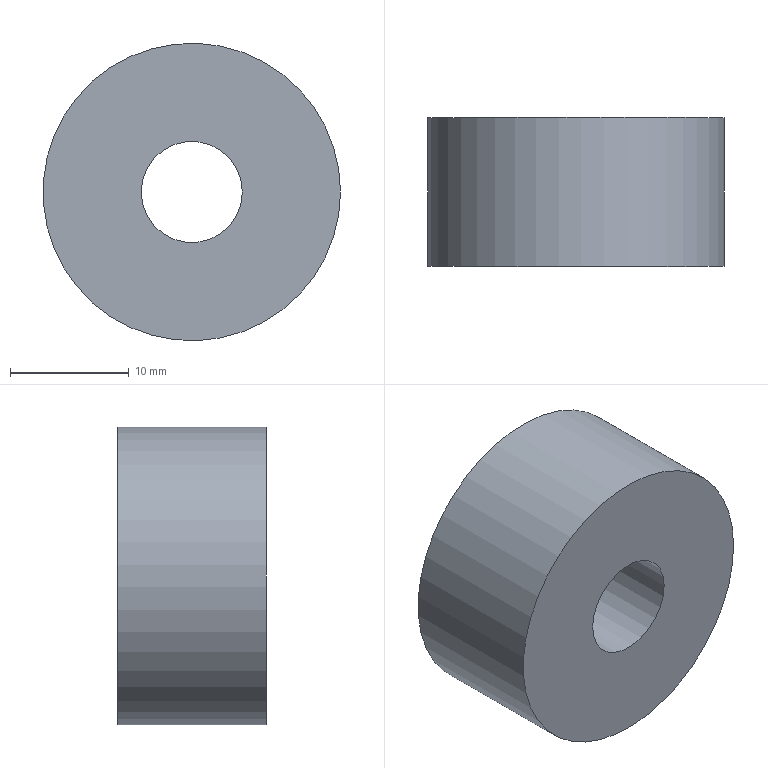Component | NX | 7_WASHER | 1 solid | 4 faces | box 25 x 12.5 x 25 mm | volume 5427 mm3 | plane 2 | cylinder 2 | commonest cylinder face diameters 25 x1 8.5 x1
STEP:
#1=CARTESIAN_POINT('',(0.,0.,0.));
#2=DIRECTION('',(0.,0.,1.));
#3=DIRECTION('',(1.,0.,0.));
#4=AXIS2_PLACEMENT_3D('',#1,#2,#3);
#5=CARTESIAN_POINT('',(6.27,26.63,14.672));
#6=VERTEX_POINT('',#5);
#7=CARTESIAN_POINT('',(2.02,26.63,14.672));
#8=DIRECTION('',(0.,-1.,0.));
#9=DIRECTION('',(1.,0.,0.));
#10=AXIS2_PLACEMENT_3D('',#7,#8,#9);
#11=CIRCLE('',#10,4.25);
#12=CARTESIAN_POINT('',(2.02,26.63,14.672));
#13=DIRECTION('',(0.,1.,0.));
#14=DIRECTION('',(1.,0.,0.));
#15=AXIS2_PLACEMENT_3D('',#12,#13,#14);
#16=PLANE('',#15);
#17=CARTESIAN_POINT('',(4.25,0.));
#18=CARTESIAN_POINT('',(4.25,-7.361));
#19=CARTESIAN_POINT('',(-2.125,-3.681));
#20=CARTESIAN_POINT('',(-8.5,-0.));
#21=CARTESIAN_POINT('',(-2.125,3.681));
#22=CARTESIAN_POINT('',(4.25,7.361));
#23=CARTESIAN_POINT('',(4.25,0.));
#24=(BOUNDED_CURVE()B_SPLINE_CURVE(2,(#17,#18,#19,#20,#21,#22,#23),.UNSPECIFIED.,.T.,.F.)B_SPLINE_CURVE_WITH_KNOTS((1,2,2,2,2,1),(-2.094,0.,2.094,4.189,6.283,8.378),.UNSPECIFIED.)CURVE()GEOMETRIC_REPRESENTATION_ITEM()RATIONAL_B_SPLINE_CURVE((1.,0.5,1.,0.5,1.,0.5,1.))REPRESENTATION_ITEM(''));
#25=(GEOMETRIC_REPRESENTATION_CONTEXT(2)PARAMETRIC_REPRESENTATION_CONTEXT()REPRESENTATION_CONTEXT('',''));
#26=DEFINITIONAL_REPRESENTATION('',(#24),#25);
#27=PCURVE('',#16,#26);
#28=CARTESIAN_POINT('',(2.02,14.13,14.672));
#29=DIRECTION('',(0.,1.,0.));
#30=DIRECTION('',(1.,0.,0.));
#31=AXIS2_PLACEMENT_3D('',#28,#29,#30);
#32=CYLINDRICAL_SURFACE('',#31,4.25);
#33=CARTESIAN_POINT('',(6.283,12.5));
#34=DIRECTION('',(-1.,0.));
#35=VECTOR('',#34,1.);
#36=LINE('',#33,#35);
#37=(GEOMETRIC_REPRESENTATION_CONTEXT(2)PARAMETRIC_REPRESENTATION_CONTEXT()REPRESENTATION_CONTEXT('',''));
#38=DEFINITIONAL_REPRESENTATION('',(#36),#37);
#39=PCURVE('',#32,#38);
#40=SURFACE_CURVE('',#11,(#27,#39),.PCURVE_S1.);
#41=EDGE_CURVE('',#6,#6,#40,.T.);
#42=ORIENTED_EDGE('',*,*,#41,.T.);
#43=EDGE_LOOP('',(#42));
#44=FACE_BOUND('',#43,.T.);
#45=CARTESIAN_POINT('',(14.52,26.63,14.672));
#46=VERTEX_POINT('',#45);
#47=CARTESIAN_POINT('',(2.02,26.63,14.672));
#48=DIRECTION('',(0.,-1.,0.));
#49=DIRECTION('',(1.,0.,0.));
#50=AXIS2_PLACEMENT_3D('',#47,#48,#49);
#51=CIRCLE('',#50,12.5);
#52=CARTESIAN_POINT('',(12.5,0.));
#53=CARTESIAN_POINT('',(12.5,-21.651));
#54=CARTESIAN_POINT('',(-6.25,-10.825));
#55=CARTESIAN_POINT('',(-25.,-0.));
#56=CARTESIAN_POINT('',(-6.25,10.825));
#57=CARTESIAN_POINT('',(12.5,21.651));
#58=CARTESIAN_POINT('',(12.5,0.));
#59=(BOUNDED_CURVE()B_SPLINE_CURVE(2,(#52,#53,#54,#55,#56,#57,#58),.UNSPECIFIED.,.T.,.F.)B_SPLINE_CURVE_WITH_KNOTS((1,2,2,2,2,1),(-2.094,0.,2.094,4.189,6.283,8.378),.UNSPECIFIED.)CURVE()GEOMETRIC_REPRESENTATION_ITEM()RATIONAL_B_SPLINE_CURVE((1.,0.5,1.,0.5,1.,0.5,1.))REPRESENTATION_ITEM(''));
#60=(GEOMETRIC_REPRESENTATION_CONTEXT(2)PARAMETRIC_REPRESENTATION_CONTEXT()REPRESENTATION_CONTEXT('',''));
#61=DEFINITIONAL_REPRESENTATION('',(#59),#60);
#62=PCURVE('',#16,#61);
#63=CARTESIAN_POINT('',(2.02,14.13,14.672));
#64=DIRECTION('',(0.,1.,0.));
#65=DIRECTION('',(1.,0.,0.));
#66=AXIS2_PLACEMENT_3D('',#63,#64,#65);
#67=CYLINDRICAL_SURFACE('',#66,12.5);
#68=CARTESIAN_POINT('',(6.283,12.5));
#69=DIRECTION('',(-1.,0.));
#70=VECTOR('',#69,1.);
#71=LINE('',#68,#70);
#72=(GEOMETRIC_REPRESENTATION_CONTEXT(2)PARAMETRIC_REPRESENTATION_CONTEXT()REPRESENTATION_CONTEXT('',''));
#73=DEFINITIONAL_REPRESENTATION('',(#71),#72);
#74=PCURVE('',#67,#73);
#75=SURFACE_CURVE('',#51,(#62,#74),.PCURVE_S1.);
#76=EDGE_CURVE('',#46,#46,#75,.T.);
#77=ORIENTED_EDGE('',*,*,#76,.F.);
#78=EDGE_LOOP('',(#77));
#79=FACE_BOUND('',#78,.T.);
#80=ADVANCED_FACE('',(#44,#79),#16,.T.);
#81=CARTESIAN_POINT('',(6.27,14.13,14.672));
#82=VERTEX_POINT('',#81);
#83=CARTESIAN_POINT('',(2.02,14.13,14.672));
#84=DIRECTION('',(0.,1.,0.));
#85=DIRECTION('',(1.,0.,0.));
#86=AXIS2_PLACEMENT_3D('',#83,#84,#85);
#87=CIRCLE('',#86,4.25);
#88=CARTESIAN_POINT('',(2.02,14.13,14.672));
#89=DIRECTION('',(0.,-1.,0.));
#90=DIRECTION('',(-1.,0.,0.));
#91=AXIS2_PLACEMENT_3D('',#88,#89,#90);
#92=PLANE('',#91);
#93=CARTESIAN_POINT('',(-4.25,0.));
#94=CARTESIAN_POINT('',(-4.25,7.361));
#95=CARTESIAN_POINT('',(2.125,3.681));
#96=CARTESIAN_POINT('',(8.5,0.));
#97=CARTESIAN_POINT('',(2.125,-3.681));
#98=CARTESIAN_POINT('',(-4.25,-7.361));
#99=CARTESIAN_POINT('',(-4.25,0.));
#100=(BOUNDED_CURVE()B_SPLINE_CURVE(2,(#93,#94,#95,#96,#97,#98,#99),.UNSPECIFIED.,.T.,.F.)B_SPLINE_CURVE_WITH_KNOTS((1,2,2,2,2,1),(-2.094,0.,2.094,4.189,6.283,8.378),.UNSPECIFIED.)CURVE()GEOMETRIC_REPRESENTATION_ITEM()RATIONAL_B_SPLINE_CURVE((1.,0.5,1.,0.5,1.,0.5,1.))REPRESENTATION_ITEM(''));
#101=(GEOMETRIC_REPRESENTATION_CONTEXT(2)PARAMETRIC_REPRESENTATION_CONTEXT()REPRESENTATION_CONTEXT('',''));
#102=DEFINITIONAL_REPRESENTATION('',(#100),#101);
#103=PCURVE('',#92,#102);
#104=CARTESIAN_POINT('',(0.,0.));
#105=DIRECTION('',(1.,0.));
#106=VECTOR('',#105,1.);
#107=LINE('',#104,#106);
#108=(GEOMETRIC_REPRESENTATION_CONTEXT(2)PARAMETRIC_REPRESENTATION_CONTEXT()REPRESENTATION_CONTEXT('',''));
#109=DEFINITIONAL_REPRESENTATION('',(#107),#108);
#110=PCURVE('',#32,#109);
#111=SURFACE_CURVE('',#87,(#103,#110),.PCURVE_S1.);
#112=EDGE_CURVE('',#82,#82,#111,.T.);
#113=ORIENTED_EDGE('',*,*,#112,.T.);
#114=EDGE_LOOP('',(#113));
#115=FACE_BOUND('',#114,.T.);
#116=CARTESIAN_POINT('',(14.52,14.13,14.672));
#117=VERTEX_POINT('',#116);
#118=CARTESIAN_POINT('',(2.02,14.13,14.672));
#119=DIRECTION('',(0.,1.,0.));
#120=DIRECTION('',(1.,0.,0.));
#121=AXIS2_PLACEMENT_3D('',#118,#119,#120);
#122=CIRCLE('',#121,12.5);
#123=CARTESIAN_POINT('',(-12.5,0.));
#124=CARTESIAN_POINT('',(-12.5,21.651));
#125=CARTESIAN_POINT('',(6.25,10.825));
#126=CARTESIAN_POINT('',(25.,0.));
#127=CARTESIAN_POINT('',(6.25,-10.825));
#128=CARTESIAN_POINT('',(-12.5,-21.651));
#129=CARTESIAN_POINT('',(-12.5,0.));
#130=(BOUNDED_CURVE()B_SPLINE_CURVE(2,(#123,#124,#125,#126,#127,#128,#129),.UNSPECIFIED.,.T.,.F.)B_SPLINE_CURVE_WITH_KNOTS((1,2,2,2,2,1),(-2.094,0.,2.094,4.189,6.283,8.378),.UNSPECIFIED.)CURVE()GEOMETRIC_REPRESENTATION_ITEM()RATIONAL_B_SPLINE_CURVE((1.,0.5,1.,0.5,1.,0.5,1.))REPRESENTATION_ITEM(''));
#131=(GEOMETRIC_REPRESENTATION_CONTEXT(2)PARAMETRIC_REPRESENTATION_CONTEXT()REPRESENTATION_CONTEXT('',''));
#132=DEFINITIONAL_REPRESENTATION('',(#130),#131);
#133=PCURVE('',#92,#132);
#134=CARTESIAN_POINT('',(0.,0.));
#135=DIRECTION('',(1.,0.));
#136=VECTOR('',#135,1.);
#137=LINE('',#134,#136);
#138=(GEOMETRIC_REPRESENTATION_CONTEXT(2)PARAMETRIC_REPRESENTATION_CONTEXT()REPRESENTATION_CONTEXT('',''));
#139=DEFINITIONAL_REPRESENTATION('',(#137),#138);
#140=PCURVE('',#67,#139);
#141=SURFACE_CURVE('',#122,(#133,#140),.PCURVE_S1.);
#142=EDGE_CURVE('',#117,#117,#141,.T.);
#143=ORIENTED_EDGE('',*,*,#142,.F.);
#144=EDGE_LOOP('',(#143));
#145=FACE_BOUND('',#144,.T.);
#146=ADVANCED_FACE('',(#115,#145),#92,.T.);
#147=ORIENTED_EDGE('',*,*,#76,.T.);
#148=CARTESIAN_POINT('',(14.52,14.13,14.672));
#149=CARTESIAN_POINT('',(14.52,26.63,14.672));
#150=B_SPLINE_CURVE_WITH_KNOTS('',1,(#148,#149),.UNSPECIFIED.,.F.,.F.,(2,2),(0.,12.5),.PIECEWISE_BEZIER_KNOTS.);
#151=CARTESIAN_POINT('',(0.,0.));
#152=DIRECTION('',(0.,1.));
#153=VECTOR('',#152,1.);
#154=LINE('',#151,#153);
#155=(GEOMETRIC_REPRESENTATION_CONTEXT(2)PARAMETRIC_REPRESENTATION_CONTEXT()REPRESENTATION_CONTEXT('',''));
#156=DEFINITIONAL_REPRESENTATION('',(#154),#155);
#157=PCURVE('',#67,#156);
#158=CARTESIAN_POINT('',(6.283,0.));
#159=DIRECTION('',(0.,1.));
#160=VECTOR('',#159,1.);
#161=LINE('',#158,#160);
#162=(GEOMETRIC_REPRESENTATION_CONTEXT(2)PARAMETRIC_REPRESENTATION_CONTEXT()REPRESENTATION_CONTEXT('',''));
#163=DEFINITIONAL_REPRESENTATION('',(#161),#162);
#164=PCURVE('',#67,#163);
#165=SEAM_CURVE('',#150,(#157,#164),.PCURVE_S1.);
#166=EDGE_CURVE('',#117,#46,#165,.T.);
#167=ORIENTED_EDGE('',*,*,#166,.F.);
#168=ORIENTED_EDGE('',*,*,#142,.T.);
#169=ORIENTED_EDGE('',*,*,#166,.T.);
#170=EDGE_LOOP('',(#147,#167,#168,#169));
#171=FACE_BOUND('',#170,.T.);
#172=ADVANCED_FACE('',(#171),#67,.T.);
#173=ORIENTED_EDGE('',*,*,#41,.T.);
#174=CARTESIAN_POINT('',(6.27,14.13,14.672));
#175=CARTESIAN_POINT('',(6.27,26.63,14.672));
#176=B_SPLINE_CURVE_WITH_KNOTS('',1,(#174,#175),.UNSPECIFIED.,.F.,.F.,(2,2),(0.,12.5),.PIECEWISE_BEZIER_KNOTS.);
#177=CARTESIAN_POINT('',(0.,0.));
#178=DIRECTION('',(0.,1.));
#179=VECTOR('',#178,1.);
#180=LINE('',#177,#179);
#181=(GEOMETRIC_REPRESENTATION_CONTEXT(2)PARAMETRIC_REPRESENTATION_CONTEXT()REPRESENTATION_CONTEXT('',''));
#182=DEFINITIONAL_REPRESENTATION('',(#180),#181);
#183=PCURVE('',#32,#182);
#184=CARTESIAN_POINT('',(6.283,0.));
#185=DIRECTION('',(0.,1.));
#186=VECTOR('',#185,1.);
#187=LINE('',#184,#186);
#188=(GEOMETRIC_REPRESENTATION_CONTEXT(2)PARAMETRIC_REPRESENTATION_CONTEXT()REPRESENTATION_CONTEXT('',''));
#189=DEFINITIONAL_REPRESENTATION('',(#187),#188);
#190=PCURVE('',#32,#189);
#191=SEAM_CURVE('',#176,(#183,#190),.PCURVE_S1.);
#192=EDGE_CURVE('',#82,#6,#191,.T.);
#193=ORIENTED_EDGE('',*,*,#192,.F.);
#194=ORIENTED_EDGE('',*,*,#112,.T.);
#195=ORIENTED_EDGE('',*,*,#192,.T.);
#196=EDGE_LOOP('',(#173,#193,#194,#195));
#197=FACE_BOUND('',#196,.F.);
#198=ADVANCED_FACE('',(#197),#32,.F.);
#199=CLOSED_SHELL('',(#80,#146,#172,#198));
#200=MANIFOLD_SOLID_BREP('',#199);
#201=(LENGTH_UNIT()NAMED_UNIT(*)SI_UNIT(.MILLI.,.METRE.));
#202=UNCERTAINTY_MEASURE_WITH_UNIT(LENGTH_MEASURE(0.00001),#201,'','');
#203=(NAMED_UNIT(*)PLANE_ANGLE_UNIT()SI_UNIT($,.RADIAN.));
#204=(NAMED_UNIT(*)SI_UNIT($,.STERADIAN.)SOLID_ANGLE_UNIT());
#205=(GEOMETRIC_REPRESENTATION_CONTEXT(3)GLOBAL_UNCERTAINTY_ASSIGNED_CONTEXT((#202))GLOBAL_UNIT_ASSIGNED_CONTEXT((#201,#203,#204))REPRESENTATION_CONTEXT('',''));
#206=ADVANCED_BREP_SHAPE_REPRESENTATION('',(#4,#200),#205);